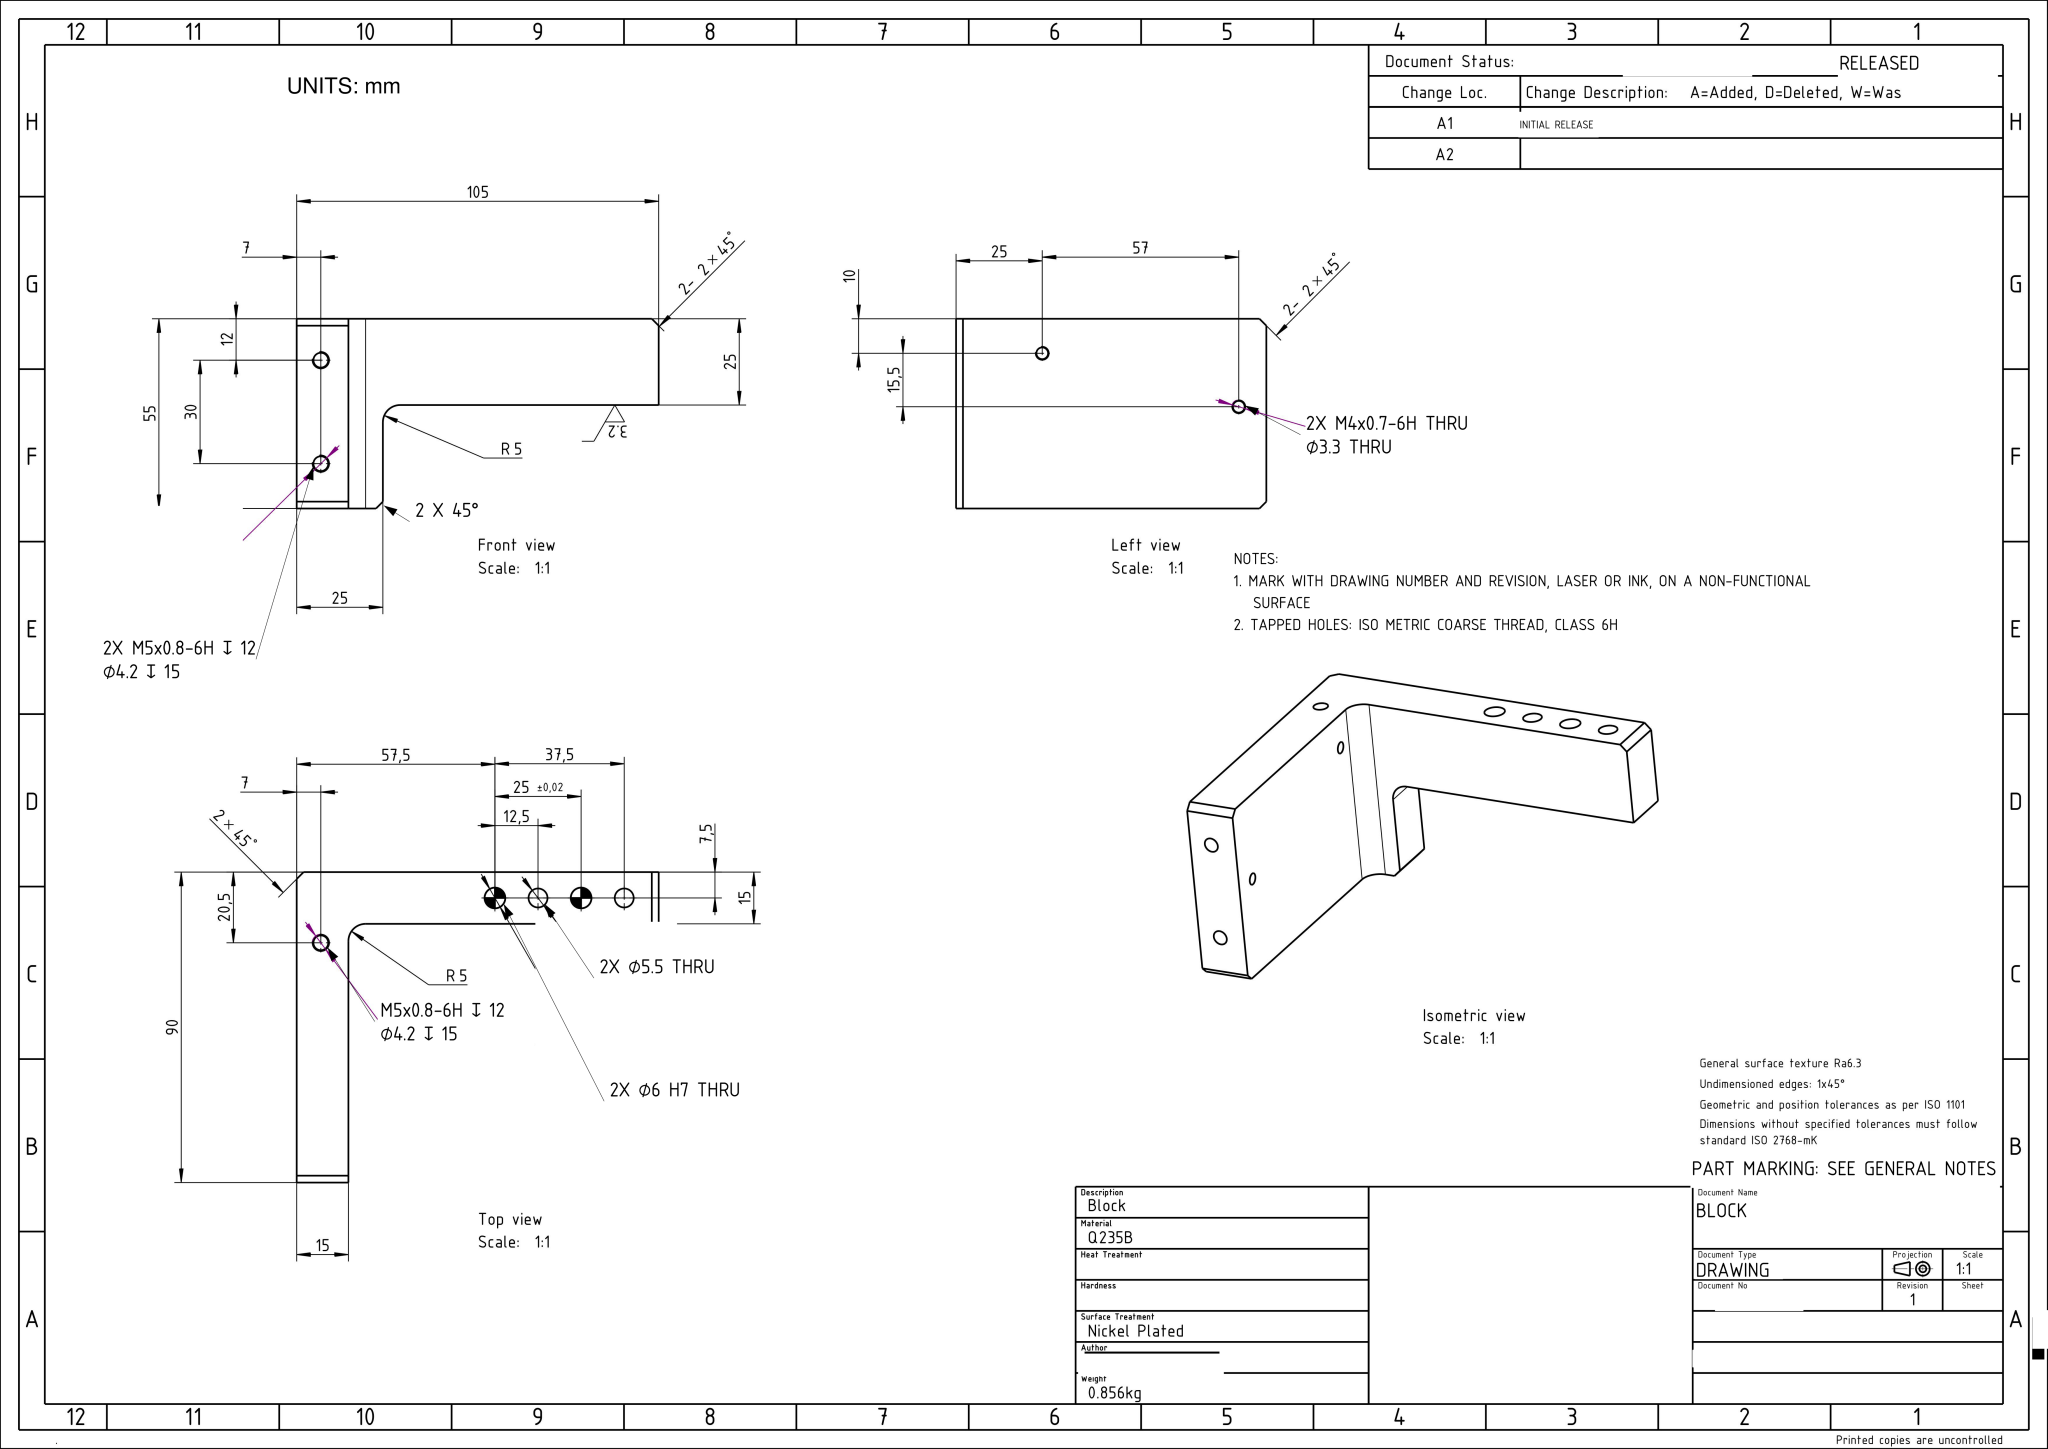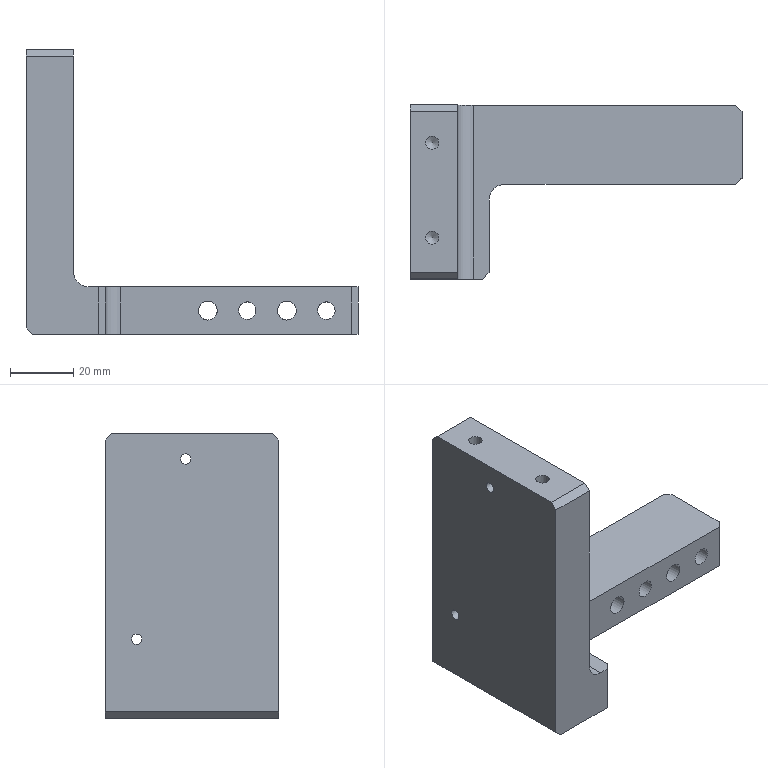Part | NX | mm | 1 solid | 30 faces | box 105 x 55 x 90 mm | volume 109116 mm3 | plane 16 | cylinder 11 | cone 3 | commonest cylinder face diameters 4.2 x3 6 x2 5.5 x2 10 x2 3.3 x2
STEP:
#1=CARTESIAN_POINT('',(0.,0.,0.));
#2=DIRECTION('',(0.,0.,1.));
#3=DIRECTION('',(1.,0.,0.));
#4=AXIS2_PLACEMENT_3D('',#1,#2,#3);
#5=(LENGTH_UNIT()NAMED_UNIT(*)SI_UNIT(.MILLI.,.METRE.));
#6=UNCERTAINTY_MEASURE_WITH_UNIT(LENGTH_MEASURE(0.00002),#5,'','');
#7=(NAMED_UNIT(*)PLANE_ANGLE_UNIT()SI_UNIT($,.RADIAN.));
#8=PLANE_ANGLE_MEASURE_WITH_UNIT(PLANE_ANGLE_MEASURE(0.01745),#7);
#9=DIMENSIONAL_EXPONENTS(0.,0.,0.,0.,0.,0.,0.);
#10=(CONVERSION_BASED_UNIT('',#8)NAMED_UNIT(#9)PLANE_ANGLE_UNIT());
#11=(NAMED_UNIT(*)SI_UNIT($,.STERADIAN.)SOLID_ANGLE_UNIT());
#12=(GEOMETRIC_REPRESENTATION_CONTEXT(3)GLOBAL_UNCERTAINTY_ASSIGNED_CONTEXT((#6))GLOBAL_UNIT_ASSIGNED_CONTEXT((#5,#10,#11))REPRESENTATION_CONTEXT('',''));
#13=SHAPE_REPRESENTATION('',(#4),#12);
#14=CARTESIAN_POINT('',(-32.5,-30.,15.));
#15=VERTEX_POINT('',#14);
#16=CARTESIAN_POINT('',(-29.5,-30.,15.));
#17=VERTEX_POINT('',#16);
#18=CARTESIAN_POINT('',(-52.5,-30.,15.));
#19=DIRECTION('',(1.,-0.,0.));
#20=VECTOR('',#19,1.);
#21=LINE('',#18,#20);
#22=EDGE_CURVE('',#15,#17,#21,.T.);
#23=ORIENTED_EDGE('',*,*,#22,.T.);
#24=CARTESIAN_POINT('',(-27.5,-28.,15.));
#25=VERTEX_POINT('',#24);
#26=CARTESIAN_POINT('',(0.25,-0.25,15.));
#27=DIRECTION('',(0.7071,0.7071,0.));
#28=VECTOR('',#27,1.);
#29=LINE('',#26,#28);
#30=EDGE_CURVE('',#17,#25,#29,.T.);
#31=ORIENTED_EDGE('',*,*,#30,.T.);
#32=CARTESIAN_POINT('',(-27.5,-5.,15.));
#33=VERTEX_POINT('',#32);
#34=CARTESIAN_POINT('',(-27.5,-30.,15.));
#35=DIRECTION('',(0.,1.,0.));
#36=VECTOR('',#35,1.);
#37=LINE('',#34,#36);
#38=EDGE_CURVE('',#25,#33,#37,.T.);
#39=ORIENTED_EDGE('',*,*,#38,.T.);
#40=CARTESIAN_POINT('',(-22.5,0.,15.));
#41=VERTEX_POINT('',#40);
#42=CARTESIAN_POINT('',(-22.5,-5.,15.));
#43=DIRECTION('',(0.,0.,-1.));
#44=DIRECTION('',(1.,0.,0.));
#45=AXIS2_PLACEMENT_3D('',#42,#43,#44);
#46=CIRCLE('',#45,5.);
#47=EDGE_CURVE('',#33,#41,#46,.T.);
#48=ORIENTED_EDGE('',*,*,#47,.T.);
#49=CARTESIAN_POINT('',(50.5,-0.,15.));
#50=VERTEX_POINT('',#49);
#51=CARTESIAN_POINT('',(-27.5,0.,15.));
#52=DIRECTION('',(1.,-0.,0.));
#53=VECTOR('',#52,1.);
#54=LINE('',#51,#53);
#55=EDGE_CURVE('',#41,#50,#54,.T.);
#56=ORIENTED_EDGE('',*,*,#55,.T.);
#57=CARTESIAN_POINT('',(52.5,2.,15.));
#58=VERTEX_POINT('',#57);
#59=CARTESIAN_POINT('',(25.25,-25.25,15.));
#60=DIRECTION('',(0.7071,0.7071,0.));
#61=VECTOR('',#60,1.);
#62=LINE('',#59,#61);
#63=EDGE_CURVE('',#50,#58,#62,.T.);
#64=ORIENTED_EDGE('',*,*,#63,.T.);
#65=CARTESIAN_POINT('',(52.5,23.,15.));
#66=VERTEX_POINT('',#65);
#67=CARTESIAN_POINT('',(52.5,-0.,15.));
#68=DIRECTION('',(0.,1.,0.));
#69=VECTOR('',#68,1.);
#70=LINE('',#67,#69);
#71=EDGE_CURVE('',#58,#66,#70,.T.);
#72=ORIENTED_EDGE('',*,*,#71,.T.);
#73=CARTESIAN_POINT('',(50.5,25.,15.));
#74=VERTEX_POINT('',#73);
#75=CARTESIAN_POINT('',(37.75,37.75,15.));
#76=DIRECTION('',(-0.7071,0.7071,0.));
#77=VECTOR('',#76,1.);
#78=LINE('',#75,#77);
#79=EDGE_CURVE('',#66,#74,#78,.T.);
#80=ORIENTED_EDGE('',*,*,#79,.T.);
#81=CARTESIAN_POINT('',(-32.5,25.,15.));
#82=VERTEX_POINT('',#81);
#83=CARTESIAN_POINT('',(52.5,25.,15.));
#84=DIRECTION('',(-1.,0.,0.));
#85=VECTOR('',#84,1.);
#86=LINE('',#83,#85);
#87=EDGE_CURVE('',#74,#82,#86,.T.);
#88=ORIENTED_EDGE('',*,*,#87,.T.);
#89=CARTESIAN_POINT('',(-32.5,0.,15.));
#90=DIRECTION('',(-0.,-1.,0.));
#91=VECTOR('',#90,1.);
#92=LINE('',#89,#91);
#93=EDGE_CURVE('',#82,#15,#92,.T.);
#94=ORIENTED_EDGE('',*,*,#93,.T.);
#95=EDGE_LOOP('',(#23,#31,#39,#48,#56,#64,#72,#80,#88,#94));
#96=FACE_OUTER_BOUND('',#95,.T.);
#97=CARTESIAN_POINT('',(0.,0.,15.));
#98=DIRECTION('',(0.,0.,1.));
#99=DIRECTION('',(1.,0.,0.));
#100=AXIS2_PLACEMENT_3D('',#97,#98,#99);
#101=PLANE('',#100);
#102=ADVANCED_FACE('',(#96),#101,.T.);
#103=CARTESIAN_POINT('',(-52.5,16.65,25.));
#104=VERTEX_POINT('',#103);
#105=CARTESIAN_POINT('',(-52.5,15.,25.));
#106=DIRECTION('',(1.,-0.,0.));
#107=DIRECTION('',(0.,1.,0.));
#108=AXIS2_PLACEMENT_3D('',#105,#106,#107);
#109=CIRCLE('',#108,1.65);
#110=EDGE_CURVE('',#104,#104,#109,.T.);
#111=ORIENTED_EDGE('',*,*,#110,.T.);
#112=EDGE_LOOP('',(#111));
#113=FACE_BOUND('',#112,.T.);
#114=CARTESIAN_POINT('',(-52.5,1.15,82.));
#115=VERTEX_POINT('',#114);
#116=CARTESIAN_POINT('',(-52.5,-0.5,82.));
#117=DIRECTION('',(1.,-0.,0.));
#118=DIRECTION('',(0.,1.,0.));
#119=AXIS2_PLACEMENT_3D('',#116,#117,#118);
#120=CIRCLE('',#119,1.65);
#121=EDGE_CURVE('',#115,#115,#120,.T.);
#122=ORIENTED_EDGE('',*,*,#121,.T.);
#123=EDGE_LOOP('',(#122));
#124=FACE_BOUND('',#123,.T.);
#125=CARTESIAN_POINT('',(-52.5,25.,88.));
#126=VERTEX_POINT('',#125);
#127=CARTESIAN_POINT('',(-52.5,25.,2.));
#128=VERTEX_POINT('',#127);
#129=CARTESIAN_POINT('',(-52.5,25.,15.));
#130=DIRECTION('',(0.,0.,-1.));
#131=VECTOR('',#130,1.);
#132=LINE('',#129,#131);
#133=EDGE_CURVE('',#126,#128,#132,.T.);
#134=ORIENTED_EDGE('',*,*,#133,.T.);
#135=CARTESIAN_POINT('',(-52.5,-30.,2.));
#136=VERTEX_POINT('',#135);
#137=CARTESIAN_POINT('',(-52.5,25.,2.));
#138=DIRECTION('',(-0.,-1.,0.));
#139=VECTOR('',#138,1.);
#140=LINE('',#137,#139);
#141=EDGE_CURVE('',#128,#136,#140,.T.);
#142=ORIENTED_EDGE('',*,*,#141,.T.);
#143=CARTESIAN_POINT('',(-52.5,-30.,88.));
#144=VERTEX_POINT('',#143);
#145=CARTESIAN_POINT('',(-52.5,-30.,15.));
#146=DIRECTION('',(0.,0.,-1.));
#147=VECTOR('',#146,1.);
#148=LINE('',#145,#147);
#149=EDGE_CURVE('',#144,#136,#148,.T.);
#150=ORIENTED_EDGE('',*,*,#149,.F.);
#151=CARTESIAN_POINT('',(-52.5,-28.,90.));
#152=VERTEX_POINT('',#151);
#153=CARTESIAN_POINT('',(-52.5,-28.,90.));
#154=DIRECTION('',(0.,0.7071,0.7071));
#155=VECTOR('',#154,1.);
#156=LINE('',#153,#155);
#157=EDGE_CURVE('',#144,#152,#156,.T.);
#158=ORIENTED_EDGE('',*,*,#157,.T.);
#159=CARTESIAN_POINT('',(-52.5,23.,90.));
#160=VERTEX_POINT('',#159);
#161=CARTESIAN_POINT('',(-52.5,25.,90.));
#162=DIRECTION('',(-0.,-1.,0.));
#163=VECTOR('',#162,1.);
#164=LINE('',#161,#163);
#165=EDGE_CURVE('',#160,#152,#164,.T.);
#166=ORIENTED_EDGE('',*,*,#165,.F.);
#167=CARTESIAN_POINT('',(-52.5,25.,88.));
#168=DIRECTION('',(0.,0.7071,-0.7071));
#169=VECTOR('',#168,1.);
#170=LINE('',#167,#169);
#171=EDGE_CURVE('',#160,#126,#170,.T.);
#172=ORIENTED_EDGE('',*,*,#171,.T.);
#173=EDGE_LOOP('',(#134,#142,#150,#158,#166,#172));
#174=FACE_BOUND('',#173,.T.);
#175=CARTESIAN_POINT('',(-52.5,25.,15.));
#176=DIRECTION('',(1.,-0.,0.));
#177=DIRECTION('',(0.,1.,0.));
#178=AXIS2_PLACEMENT_3D('',#175,#176,#177);
#179=PLANE('',#178);
#180=ADVANCED_FACE('',(#113,#124,#174),#179,.F.);
#181=CARTESIAN_POINT('',(-50.5,-30.,0.));
#182=VERTEX_POINT('',#181);
#183=CARTESIAN_POINT('',(-29.5,-30.,0.));
#184=VERTEX_POINT('',#183);
#185=CARTESIAN_POINT('',(-52.5,-30.,0.));
#186=DIRECTION('',(1.,-0.,0.));
#187=VECTOR('',#186,1.);
#188=LINE('',#185,#187);
#189=EDGE_CURVE('',#182,#184,#188,.T.);
#190=ORIENTED_EDGE('',*,*,#189,.T.);
#191=CARTESIAN_POINT('',(-29.5,-30.,15.));
#192=DIRECTION('',(0.,0.,1.));
#193=VECTOR('',#192,1.);
#194=LINE('',#191,#193);
#195=EDGE_CURVE('',#184,#17,#194,.T.);
#196=ORIENTED_EDGE('',*,*,#195,.T.);
#197=ORIENTED_EDGE('',*,*,#22,.F.);
#198=CARTESIAN_POINT('',(-37.5,-30.,20.));
#199=VERTEX_POINT('',#198);
#200=CARTESIAN_POINT('',(-32.5,-30.,20.));
#201=DIRECTION('',(0.,1.,0.));
#202=DIRECTION('',(-1.,0.,0.));
#203=AXIS2_PLACEMENT_3D('',#200,#201,#202);
#204=CIRCLE('',#203,5.);
#205=EDGE_CURVE('',#15,#199,#204,.T.);
#206=ORIENTED_EDGE('',*,*,#205,.T.);
#207=CARTESIAN_POINT('',(-37.5,-30.,88.));
#208=VERTEX_POINT('',#207);
#209=CARTESIAN_POINT('',(-37.5,-30.,15.));
#210=DIRECTION('',(0.,0.,1.));
#211=VECTOR('',#210,1.);
#212=LINE('',#209,#211);
#213=EDGE_CURVE('',#199,#208,#212,.T.);
#214=ORIENTED_EDGE('',*,*,#213,.T.);
#215=CARTESIAN_POINT('',(-52.5,-30.,88.));
#216=DIRECTION('',(-1.,0.,0.));
#217=VECTOR('',#216,1.);
#218=LINE('',#215,#217);
#219=EDGE_CURVE('',#208,#144,#218,.T.);
#220=ORIENTED_EDGE('',*,*,#219,.T.);
#221=ORIENTED_EDGE('',*,*,#149,.T.);
#222=CARTESIAN_POINT('',(-52.5,-30.,2.));
#223=DIRECTION('',(0.7071,-0.,-0.7071));
#224=VECTOR('',#223,1.);
#225=LINE('',#222,#224);
#226=EDGE_CURVE('',#136,#182,#225,.T.);
#227=ORIENTED_EDGE('',*,*,#226,.T.);
#228=EDGE_LOOP('',(#190,#196,#197,#206,#214,#220,#221,#227));
#229=FACE_OUTER_BOUND('',#228,.T.);
#230=CARTESIAN_POINT('',(-52.5,-30.,15.));
#231=DIRECTION('',(0.,1.,0.));
#232=DIRECTION('',(-1.,0.,0.));
#233=AXIS2_PLACEMENT_3D('',#230,#231,#232);
#234=PLANE('',#233);
#235=ADVANCED_FACE('',(#229),#234,.F.);
#236=ORIENTED_EDGE('',*,*,#38,.F.);
#237=CARTESIAN_POINT('',(-27.5,-28.,0.));
#238=VERTEX_POINT('',#237);
#239=CARTESIAN_POINT('',(-27.5,-28.,15.));
#240=DIRECTION('',(0.,0.,-1.));
#241=VECTOR('',#240,1.);
#242=LINE('',#239,#241);
#243=EDGE_CURVE('',#25,#238,#242,.T.);
#244=ORIENTED_EDGE('',*,*,#243,.T.);
#245=CARTESIAN_POINT('',(-27.5,-5.,0.));
#246=VERTEX_POINT('',#245);
#247=CARTESIAN_POINT('',(-27.5,-30.,0.));
#248=DIRECTION('',(0.,1.,0.));
#249=VECTOR('',#248,1.);
#250=LINE('',#247,#249);
#251=EDGE_CURVE('',#238,#246,#250,.T.);
#252=ORIENTED_EDGE('',*,*,#251,.T.);
#253=CARTESIAN_POINT('',(-27.5,-5.,15.));
#254=DIRECTION('',(0.,0.,1.));
#255=VECTOR('',#254,1.);
#256=LINE('',#253,#255);
#257=EDGE_CURVE('',#246,#33,#256,.T.);
#258=ORIENTED_EDGE('',*,*,#257,.T.);
#259=EDGE_LOOP('',(#236,#244,#252,#258));
#260=FACE_OUTER_BOUND('',#259,.T.);
#261=CARTESIAN_POINT('',(-27.5,-30.,15.));
#262=DIRECTION('',(-1.,0.,0.));
#263=DIRECTION('',(0.,0.,1.));
#264=AXIS2_PLACEMENT_3D('',#261,#262,#263);
#265=PLANE('',#264);
#266=ADVANCED_FACE('',(#260),#265,.F.);
#267=CARTESIAN_POINT('',(39.75,-0.,7.5));
#268=VERTEX_POINT('',#267);
#269=CARTESIAN_POINT('',(42.5,-0.,7.5));
#270=DIRECTION('',(0.,1.,0.));
#271=DIRECTION('',(-1.,0.,0.));
#272=AXIS2_PLACEMENT_3D('',#269,#270,#271);
#273=CIRCLE('',#272,2.75);
#274=EDGE_CURVE('',#268,#268,#273,.T.);
#275=ORIENTED_EDGE('',*,*,#274,.T.);
#276=EDGE_LOOP('',(#275));
#277=FACE_BOUND('',#276,.T.);
#278=CARTESIAN_POINT('',(14.75,-0.,7.5));
#279=VERTEX_POINT('',#278);
#280=CARTESIAN_POINT('',(17.5,-0.,7.5));
#281=DIRECTION('',(0.,1.,0.));
#282=DIRECTION('',(-1.,0.,0.));
#283=AXIS2_PLACEMENT_3D('',#280,#281,#282);
#284=CIRCLE('',#283,2.75);
#285=EDGE_CURVE('',#279,#279,#284,.T.);
#286=ORIENTED_EDGE('',*,*,#285,.T.);
#287=EDGE_LOOP('',(#286));
#288=FACE_BOUND('',#287,.T.);
#289=CARTESIAN_POINT('',(27.,-0.,7.5));
#290=VERTEX_POINT('',#289);
#291=CARTESIAN_POINT('',(30.,-0.,7.5));
#292=DIRECTION('',(0.,1.,0.));
#293=DIRECTION('',(-1.,0.,0.));
#294=AXIS2_PLACEMENT_3D('',#291,#292,#293);
#295=CIRCLE('',#294,3.);
#296=EDGE_CURVE('',#290,#290,#295,.T.);
#297=ORIENTED_EDGE('',*,*,#296,.T.);
#298=EDGE_LOOP('',(#297));
#299=FACE_BOUND('',#298,.T.);
#300=CARTESIAN_POINT('',(2.,-0.,7.5));
#301=VERTEX_POINT('',#300);
#302=CARTESIAN_POINT('',(5.,-0.,7.5));
#303=DIRECTION('',(0.,1.,0.));
#304=DIRECTION('',(-1.,0.,0.));
#305=AXIS2_PLACEMENT_3D('',#302,#303,#304);
#306=CIRCLE('',#305,3.);
#307=EDGE_CURVE('',#301,#301,#306,.T.);
#308=ORIENTED_EDGE('',*,*,#307,.T.);
#309=EDGE_LOOP('',(#308));
#310=FACE_BOUND('',#309,.T.);
#311=CARTESIAN_POINT('',(-22.5,0.,0.));
#312=VERTEX_POINT('',#311);
#313=CARTESIAN_POINT('',(50.5,-0.,0.));
#314=VERTEX_POINT('',#313);
#315=CARTESIAN_POINT('',(-27.5,0.,0.));
#316=DIRECTION('',(1.,-0.,0.));
#317=VECTOR('',#316,1.);
#318=LINE('',#315,#317);
#319=EDGE_CURVE('',#312,#314,#318,.T.);
#320=ORIENTED_EDGE('',*,*,#319,.T.);
#321=CARTESIAN_POINT('',(50.5,-0.,15.));
#322=DIRECTION('',(0.,0.,1.));
#323=VECTOR('',#322,1.);
#324=LINE('',#321,#323);
#325=EDGE_CURVE('',#314,#50,#324,.T.);
#326=ORIENTED_EDGE('',*,*,#325,.T.);
#327=ORIENTED_EDGE('',*,*,#55,.F.);
#328=CARTESIAN_POINT('',(-22.5,0.,0.));
#329=DIRECTION('',(0.,0.,-1.));
#330=VECTOR('',#329,1.);
#331=LINE('',#328,#330);
#332=EDGE_CURVE('',#41,#312,#331,.T.);
#333=ORIENTED_EDGE('',*,*,#332,.T.);
#334=EDGE_LOOP('',(#320,#326,#327,#333));
#335=FACE_BOUND('',#334,.T.);
#336=CARTESIAN_POINT('',(-27.5,0.,15.));
#337=DIRECTION('',(0.,1.,0.));
#338=DIRECTION('',(-1.,0.,0.));
#339=AXIS2_PLACEMENT_3D('',#336,#337,#338);
#340=PLANE('',#339);
#341=ADVANCED_FACE('',(#277,#288,#299,#310,#335),#340,.F.);
#342=CARTESIAN_POINT('',(52.5,2.,0.));
#343=VERTEX_POINT('',#342);
#344=CARTESIAN_POINT('',(52.5,23.,0.));
#345=VERTEX_POINT('',#344);
#346=CARTESIAN_POINT('',(52.5,-0.,0.));
#347=DIRECTION('',(0.,1.,0.));
#348=VECTOR('',#347,1.);
#349=LINE('',#346,#348);
#350=EDGE_CURVE('',#343,#345,#349,.T.);
#351=ORIENTED_EDGE('',*,*,#350,.T.);
#352=CARTESIAN_POINT('',(52.5,23.,15.));
#353=DIRECTION('',(0.,0.,1.));
#354=VECTOR('',#353,1.);
#355=LINE('',#352,#354);
#356=EDGE_CURVE('',#345,#66,#355,.T.);
#357=ORIENTED_EDGE('',*,*,#356,.T.);
#358=ORIENTED_EDGE('',*,*,#71,.F.);
#359=CARTESIAN_POINT('',(52.5,2.,15.));
#360=DIRECTION('',(0.,0.,-1.));
#361=VECTOR('',#360,1.);
#362=LINE('',#359,#361);
#363=EDGE_CURVE('',#58,#343,#362,.T.);
#364=ORIENTED_EDGE('',*,*,#363,.T.);
#365=EDGE_LOOP('',(#351,#357,#358,#364));
#366=FACE_OUTER_BOUND('',#365,.T.);
#367=CARTESIAN_POINT('',(52.5,-0.,15.));
#368=DIRECTION('',(-1.,0.,0.));
#369=DIRECTION('',(0.,0.,1.));
#370=AXIS2_PLACEMENT_3D('',#367,#368,#369);
#371=PLANE('',#370);
#372=ADVANCED_FACE('',(#366),#371,.F.);
#373=CARTESIAN_POINT('',(42.5,25.,4.75));
#374=VERTEX_POINT('',#373);
#375=CARTESIAN_POINT('',(42.5,25.,7.5));
#376=DIRECTION('',(0.,-1.,0.));
#377=DIRECTION('',(0.,0.,-1.));
#378=AXIS2_PLACEMENT_3D('',#375,#376,#377);
#379=CIRCLE('',#378,2.75);
#380=EDGE_CURVE('',#374,#374,#379,.T.);
#381=ORIENTED_EDGE('',*,*,#380,.T.);
#382=EDGE_LOOP('',(#381));
#383=FACE_BOUND('',#382,.T.);
#384=CARTESIAN_POINT('',(17.5,25.,4.75));
#385=VERTEX_POINT('',#384);
#386=CARTESIAN_POINT('',(17.5,25.,7.5));
#387=DIRECTION('',(0.,-1.,0.));
#388=DIRECTION('',(0.,0.,-1.));
#389=AXIS2_PLACEMENT_3D('',#386,#387,#388);
#390=CIRCLE('',#389,2.75);
#391=EDGE_CURVE('',#385,#385,#390,.T.);
#392=ORIENTED_EDGE('',*,*,#391,.T.);
#393=EDGE_LOOP('',(#392));
#394=FACE_BOUND('',#393,.T.);
#395=CARTESIAN_POINT('',(30.,25.,4.5));
#396=VERTEX_POINT('',#395);
#397=CARTESIAN_POINT('',(30.,25.,7.5));
#398=DIRECTION('',(0.,-1.,0.));
#399=DIRECTION('',(0.,0.,-1.));
#400=AXIS2_PLACEMENT_3D('',#397,#398,#399);
#401=CIRCLE('',#400,3.);
#402=EDGE_CURVE('',#396,#396,#401,.T.);
#403=ORIENTED_EDGE('',*,*,#402,.T.);
#404=EDGE_LOOP('',(#403));
#405=FACE_BOUND('',#404,.T.);
#406=CARTESIAN_POINT('',(5.,25.,4.5));
#407=VERTEX_POINT('',#406);
#408=CARTESIAN_POINT('',(5.,25.,7.5));
#409=DIRECTION('',(0.,-1.,0.));
#410=DIRECTION('',(0.,0.,-1.));
#411=AXIS2_PLACEMENT_3D('',#408,#409,#410);
#412=CIRCLE('',#411,3.);
#413=EDGE_CURVE('',#407,#407,#412,.T.);
#414=ORIENTED_EDGE('',*,*,#413,.T.);
#415=EDGE_LOOP('',(#414));
#416=FACE_BOUND('',#415,.T.);
#417=CARTESIAN_POINT('',(-45.5,25.,18.4));
#418=VERTEX_POINT('',#417);
#419=CARTESIAN_POINT('',(-45.5,25.,20.5));
#420=DIRECTION('',(0.,-1.,0.));
#421=DIRECTION('',(0.,0.,-1.));
#422=AXIS2_PLACEMENT_3D('',#419,#420,#421);
#423=CIRCLE('',#422,2.1);
#424=EDGE_CURVE('',#418,#418,#423,.T.);
#425=ORIENTED_EDGE('',*,*,#424,.T.);
#426=EDGE_LOOP('',(#425));
#427=FACE_BOUND('',#426,.T.);
#428=CARTESIAN_POINT('',(50.5,25.,0.));
#429=VERTEX_POINT('',#428);
#430=CARTESIAN_POINT('',(-50.5,25.,0.));
#431=VERTEX_POINT('',#430);
#432=CARTESIAN_POINT('',(52.5,25.,0.));
#433=DIRECTION('',(-1.,0.,0.));
#434=VECTOR('',#433,1.);
#435=LINE('',#432,#434);
#436=EDGE_CURVE('',#429,#431,#435,.T.);
#437=ORIENTED_EDGE('',*,*,#436,.T.);
#438=CARTESIAN_POINT('',(-52.5,25.,2.));
#439=DIRECTION('',(-0.7071,0.,0.7071));
#440=VECTOR('',#439,1.);
#441=LINE('',#438,#440);
#442=EDGE_CURVE('',#431,#128,#441,.T.);
#443=ORIENTED_EDGE('',*,*,#442,.T.);
#444=ORIENTED_EDGE('',*,*,#133,.F.);
#445=CARTESIAN_POINT('',(-37.5,25.,88.));
#446=VERTEX_POINT('',#445);
#447=CARTESIAN_POINT('',(52.5,25.,88.));
#448=DIRECTION('',(1.,0.,0.));
#449=VECTOR('',#448,1.);
#450=LINE('',#447,#449);
#451=EDGE_CURVE('',#126,#446,#450,.T.);
#452=ORIENTED_EDGE('',*,*,#451,.T.);
#453=CARTESIAN_POINT('',(-37.5,25.,20.));
#454=VERTEX_POINT('',#453);
#455=CARTESIAN_POINT('',(-37.5,25.,15.));
#456=DIRECTION('',(0.,0.,1.));
#457=VECTOR('',#456,1.);
#458=LINE('',#455,#457);
#459=EDGE_CURVE('',#454,#446,#458,.T.);
#460=ORIENTED_EDGE('',*,*,#459,.F.);
#461=CARTESIAN_POINT('',(-32.5,25.,20.));
#462=DIRECTION('',(0.,-1.,0.));
#463=DIRECTION('',(0.,0.,-1.));
#464=AXIS2_PLACEMENT_3D('',#461,#462,#463);
#465=CIRCLE('',#464,5.);
#466=EDGE_CURVE('',#454,#82,#465,.T.);
#467=ORIENTED_EDGE('',*,*,#466,.T.);
#468=ORIENTED_EDGE('',*,*,#87,.F.);
#469=CARTESIAN_POINT('',(50.5,25.,15.));
#470=DIRECTION('',(0.,0.,-1.));
#471=VECTOR('',#470,1.);
#472=LINE('',#469,#471);
#473=EDGE_CURVE('',#74,#429,#472,.T.);
#474=ORIENTED_EDGE('',*,*,#473,.T.);
#475=EDGE_LOOP('',(#437,#443,#444,#452,#460,#467,#468,#474));
#476=FACE_BOUND('',#475,.T.);
#477=CARTESIAN_POINT('',(52.5,25.,15.));
#478=DIRECTION('',(0.,-1.,0.));
#479=DIRECTION('',(0.,0.,-1.));
#480=AXIS2_PLACEMENT_3D('',#477,#478,#479);
#481=PLANE('',#480);
#482=ADVANCED_FACE('',(#383,#394,#405,#416,#427,#476),#481,.F.);
#483=ORIENTED_EDGE('',*,*,#251,.F.);
#484=CARTESIAN_POINT('',(-27.5,-28.,0.));
#485=DIRECTION('',(-0.7071,-0.7071,0.));
#486=VECTOR('',#485,1.);
#487=LINE('',#484,#486);
#488=EDGE_CURVE('',#238,#184,#487,.T.);
#489=ORIENTED_EDGE('',*,*,#488,.T.);
#490=ORIENTED_EDGE('',*,*,#189,.F.);
#491=CARTESIAN_POINT('',(-50.5,0.,0.));
#492=DIRECTION('',(0.,1.,0.));
#493=VECTOR('',#492,1.);
#494=LINE('',#491,#493);
#495=EDGE_CURVE('',#182,#431,#494,.T.);
#496=ORIENTED_EDGE('',*,*,#495,.T.);
#497=ORIENTED_EDGE('',*,*,#436,.F.);
#498=CARTESIAN_POINT('',(50.5,25.,0.));
#499=DIRECTION('',(0.7071,-0.7071,0.));
#500=VECTOR('',#499,1.);
#501=LINE('',#498,#500);
#502=EDGE_CURVE('',#429,#345,#501,.T.);
#503=ORIENTED_EDGE('',*,*,#502,.T.);
#504=ORIENTED_EDGE('',*,*,#350,.F.);
#505=CARTESIAN_POINT('',(52.5,2.,0.));
#506=DIRECTION('',(-0.7071,-0.7071,0.));
#507=VECTOR('',#506,1.);
#508=LINE('',#505,#507);
#509=EDGE_CURVE('',#343,#314,#508,.T.);
#510=ORIENTED_EDGE('',*,*,#509,.T.);
#511=ORIENTED_EDGE('',*,*,#319,.F.);
#512=CARTESIAN_POINT('',(-22.5,-5.,0.));
#513=DIRECTION('',(0.,0.,1.));
#514=DIRECTION('',(1.,0.,0.));
#515=AXIS2_PLACEMENT_3D('',#512,#513,#514);
#516=CIRCLE('',#515,5.);
#517=EDGE_CURVE('',#312,#246,#516,.T.);
#518=ORIENTED_EDGE('',*,*,#517,.T.);
#519=EDGE_LOOP('',(#483,#489,#490,#496,#497,#503,#504,#510,#511,#518));
#520=FACE_OUTER_BOUND('',#519,.T.);
#521=CARTESIAN_POINT('',(0.,0.,0.));
#522=DIRECTION('',(0.,0.,1.));
#523=DIRECTION('',(1.,0.,0.));
#524=AXIS2_PLACEMENT_3D('',#521,#522,#523);
#525=PLANE('',#524);
#526=ADVANCED_FACE('',(#520),#525,.F.);
#527=CARTESIAN_POINT('',(-47.6,13.,90.));
#528=VERTEX_POINT('',#527);
#529=CARTESIAN_POINT('',(-45.5,13.,90.));
#530=DIRECTION('',(0.,0.,-1.));
#531=DIRECTION('',(-1.,0.,0.));
#532=AXIS2_PLACEMENT_3D('',#529,#530,#531);
#533=CIRCLE('',#532,2.1);
#534=EDGE_CURVE('',#528,#528,#533,.T.);
#535=ORIENTED_EDGE('',*,*,#534,.T.);
#536=EDGE_LOOP('',(#535));
#537=FACE_BOUND('',#536,.T.);
#538=CARTESIAN_POINT('',(-47.6,-17.,90.));
#539=VERTEX_POINT('',#538);
#540=CARTESIAN_POINT('',(-45.5,-17.,90.));
#541=DIRECTION('',(0.,0.,-1.));
#542=DIRECTION('',(-1.,0.,0.));
#543=AXIS2_PLACEMENT_3D('',#540,#541,#542);
#544=CIRCLE('',#543,2.1);
#545=EDGE_CURVE('',#539,#539,#544,.T.);
#546=ORIENTED_EDGE('',*,*,#545,.T.);
#547=EDGE_LOOP('',(#546));
#548=FACE_BOUND('',#547,.T.);
#549=CARTESIAN_POINT('',(-37.5,23.,90.));
#550=VERTEX_POINT('',#549);
#551=CARTESIAN_POINT('',(-37.5,-28.,90.));
#552=VERTEX_POINT('',#551);
#553=CARTESIAN_POINT('',(-37.5,25.,90.));
#554=DIRECTION('',(-0.,-1.,0.));
#555=VECTOR('',#554,1.);
#556=LINE('',#553,#555);
#557=EDGE_CURVE('',#550,#552,#556,.T.);
#558=ORIENTED_EDGE('',*,*,#557,.F.);
#559=CARTESIAN_POINT('',(-52.5,23.,90.));
#560=DIRECTION('',(-1.,0.,0.));
#561=VECTOR('',#560,1.);
#562=LINE('',#559,#561);
#563=EDGE_CURVE('',#550,#160,#562,.T.);
#564=ORIENTED_EDGE('',*,*,#563,.T.);
#565=ORIENTED_EDGE('',*,*,#165,.T.);
#566=CARTESIAN_POINT('',(-52.5,-28.,90.));
#567=DIRECTION('',(1.,-0.,0.));
#568=VECTOR('',#567,1.);
#569=LINE('',#566,#568);
#570=EDGE_CURVE('',#152,#552,#569,.T.);
#571=ORIENTED_EDGE('',*,*,#570,.T.);
#572=EDGE_LOOP('',(#558,#564,#565,#571));
#573=FACE_BOUND('',#572,.T.);
#574=CARTESIAN_POINT('',(-52.5,25.,90.));
#575=DIRECTION('',(0.,0.,-1.));
#576=DIRECTION('',(-0.,-1.,0.));
#577=AXIS2_PLACEMENT_3D('',#574,#575,#576);
#578=PLANE('',#577);
#579=ADVANCED_FACE('',(#537,#548,#573),#578,.F.);
#580=CARTESIAN_POINT('',(-37.5,13.35,25.));
#581=VERTEX_POINT('',#580);
#582=CARTESIAN_POINT('',(-37.5,15.,25.));
#583=DIRECTION('',(-1.,0.,0.));
#584=DIRECTION('',(0.,-1.,0.));
#585=AXIS2_PLACEMENT_3D('',#582,#583,#584);
#586=CIRCLE('',#585,1.65);
#587=EDGE_CURVE('',#581,#581,#586,.T.);
#588=ORIENTED_EDGE('',*,*,#587,.T.);
#589=EDGE_LOOP('',(#588));
#590=FACE_BOUND('',#589,.T.);
#591=CARTESIAN_POINT('',(-37.5,-2.15,82.));
#592=VERTEX_POINT('',#591);
#593=CARTESIAN_POINT('',(-37.5,-0.5,82.));
#594=DIRECTION('',(-1.,0.,0.));
#595=DIRECTION('',(0.,-1.,0.));
#596=AXIS2_PLACEMENT_3D('',#593,#594,#595);
#597=CIRCLE('',#596,1.65);
#598=EDGE_CURVE('',#592,#592,#597,.T.);
#599=ORIENTED_EDGE('',*,*,#598,.T.);
#600=EDGE_LOOP('',(#599));
#601=FACE_BOUND('',#600,.T.);
#602=ORIENTED_EDGE('',*,*,#459,.T.);
#603=CARTESIAN_POINT('',(-37.5,25.,88.));
#604=DIRECTION('',(-0.,-0.7071,0.7071));
#605=VECTOR('',#604,1.);
#606=LINE('',#603,#605);
#607=EDGE_CURVE('',#446,#550,#606,.T.);
#608=ORIENTED_EDGE('',*,*,#607,.T.);
#609=ORIENTED_EDGE('',*,*,#557,.T.);
#610=CARTESIAN_POINT('',(-37.5,-28.,90.));
#611=DIRECTION('',(-0.,-0.7071,-0.7071));
#612=VECTOR('',#611,1.);
#613=LINE('',#610,#612);
#614=EDGE_CURVE('',#552,#208,#613,.T.);
#615=ORIENTED_EDGE('',*,*,#614,.T.);
#616=ORIENTED_EDGE('',*,*,#213,.F.);
#617=CARTESIAN_POINT('',(-37.5,25.,20.));
#618=DIRECTION('',(0.,1.,0.));
#619=VECTOR('',#618,1.);
#620=LINE('',#617,#619);
#621=EDGE_CURVE('',#199,#454,#620,.T.);
#622=ORIENTED_EDGE('',*,*,#621,.T.);
#623=EDGE_LOOP('',(#602,#608,#609,#615,#616,#622));
#624=FACE_BOUND('',#623,.T.);
#625=CARTESIAN_POINT('',(-37.5,25.,15.));
#626=DIRECTION('',(-1.,0.,0.));
#627=DIRECTION('',(-0.,-1.,0.));
#628=AXIS2_PLACEMENT_3D('',#625,#626,#627);
#629=PLANE('',#628);
#630=ADVANCED_FACE('',(#590,#601,#624),#629,.F.);
#631=CARTESIAN_POINT('',(-47.6,-17.,75.));
#632=VERTEX_POINT('',#631);
#633=CARTESIAN_POINT('',(-45.5,-17.,75.));
#634=DIRECTION('',(0.,0.,1.));
#635=DIRECTION('',(-1.,0.,0.));
#636=AXIS2_PLACEMENT_3D('',#633,#634,#635);
#637=CIRCLE('',#636,2.1);
#638=EDGE_CURVE('',#632,#632,#637,.T.);
#639=ORIENTED_EDGE('',*,*,#638,.T.);
#640=EDGE_LOOP('',(#639));
#641=FACE_BOUND('',#640,.T.);
#642=CARTESIAN_POINT('',(-45.5,-17.,73.738));
#643=VERTEX_POINT('',#642);
#644=VERTEX_LOOP('',#643);
#645=FACE_BOUND('',#644,.T.);
#646=CARTESIAN_POINT('',(-45.5,-17.,75.));
#647=DIRECTION('',(0.,0.,1.));
#648=DIRECTION('',(1.,0.,-0.));
#649=AXIS2_PLACEMENT_3D('',#646,#647,#648);
#650=CONICAL_SURFACE('',#649,2.1,59.);
#651=ADVANCED_FACE('',(#641,#645),#650,.F.);
#652=ORIENTED_EDGE('',*,*,#638,.F.);
#653=EDGE_LOOP('',(#652));
#654=FACE_BOUND('',#653,.T.);
#655=ORIENTED_EDGE('',*,*,#545,.F.);
#656=EDGE_LOOP('',(#655));
#657=FACE_BOUND('',#656,.T.);
#658=CARTESIAN_POINT('',(-45.5,-17.,90.));
#659=DIRECTION('',(0.,0.,-1.));
#660=DIRECTION('',(-1.,0.,0.));
#661=AXIS2_PLACEMENT_3D('',#658,#659,#660);
#662=CYLINDRICAL_SURFACE('',#661,2.1);
#663=ADVANCED_FACE('',(#654,#657),#662,.F.);
#664=CARTESIAN_POINT('',(-47.6,13.,75.));
#665=VERTEX_POINT('',#664);
#666=CARTESIAN_POINT('',(-45.5,13.,75.));
#667=DIRECTION('',(0.,0.,1.));
#668=DIRECTION('',(-1.,0.,0.));
#669=AXIS2_PLACEMENT_3D('',#666,#667,#668);
#670=CIRCLE('',#669,2.1);
#671=EDGE_CURVE('',#665,#665,#670,.T.);
#672=ORIENTED_EDGE('',*,*,#671,.T.);
#673=EDGE_LOOP('',(#672));
#674=FACE_BOUND('',#673,.T.);
#675=CARTESIAN_POINT('',(-45.5,13.,73.738));
#676=VERTEX_POINT('',#675);
#677=VERTEX_LOOP('',#676);
#678=FACE_BOUND('',#677,.T.);
#679=CARTESIAN_POINT('',(-45.5,13.,75.));
#680=DIRECTION('',(0.,0.,1.));
#681=DIRECTION('',(1.,0.,-0.));
#682=AXIS2_PLACEMENT_3D('',#679,#680,#681);
#683=CONICAL_SURFACE('',#682,2.1,59.);
#684=ADVANCED_FACE('',(#674,#678),#683,.F.);
#685=ORIENTED_EDGE('',*,*,#671,.F.);
#686=EDGE_LOOP('',(#685));
#687=FACE_BOUND('',#686,.T.);
#688=ORIENTED_EDGE('',*,*,#534,.F.);
#689=EDGE_LOOP('',(#688));
#690=FACE_BOUND('',#689,.T.);
#691=CARTESIAN_POINT('',(-45.5,13.,90.));
#692=DIRECTION('',(0.,0.,-1.));
#693=DIRECTION('',(-1.,0.,0.));
#694=AXIS2_PLACEMENT_3D('',#691,#692,#693);
#695=CYLINDRICAL_SURFACE('',#694,2.1);
#696=ADVANCED_FACE('',(#687,#690),#695,.F.);
#697=CARTESIAN_POINT('',(-45.5,10.,18.4));
#698=VERTEX_POINT('',#697);
#699=CARTESIAN_POINT('',(-45.5,10.,20.5));
#700=DIRECTION('',(0.,1.,0.));
#701=DIRECTION('',(0.,0.,-1.));
#702=AXIS2_PLACEMENT_3D('',#699,#700,#701);
#703=CIRCLE('',#702,2.1);
#704=EDGE_CURVE('',#698,#698,#703,.T.);
#705=ORIENTED_EDGE('',*,*,#704,.T.);
#706=EDGE_LOOP('',(#705));
#707=FACE_BOUND('',#706,.T.);
#708=CARTESIAN_POINT('',(-45.5,8.738,20.5));
#709=VERTEX_POINT('',#708);
#710=VERTEX_LOOP('',#709);
#711=FACE_BOUND('',#710,.T.);
#712=CARTESIAN_POINT('',(-45.5,10.,20.5));
#713=DIRECTION('',(0.,1.,0.));
#714=DIRECTION('',(0.,-0.,1.));
#715=AXIS2_PLACEMENT_3D('',#712,#713,#714);
#716=CONICAL_SURFACE('',#715,2.1,59.);
#717=ADVANCED_FACE('',(#707,#711),#716,.F.);
#718=ORIENTED_EDGE('',*,*,#704,.F.);
#719=EDGE_LOOP('',(#718));
#720=FACE_BOUND('',#719,.T.);
#721=ORIENTED_EDGE('',*,*,#424,.F.);
#722=EDGE_LOOP('',(#721));
#723=FACE_BOUND('',#722,.T.);
#724=CARTESIAN_POINT('',(-45.5,25.,20.5));
#725=DIRECTION('',(0.,-1.,0.));
#726=DIRECTION('',(0.,0.,-1.));
#727=AXIS2_PLACEMENT_3D('',#724,#725,#726);
#728=CYLINDRICAL_SURFACE('',#727,2.1);
#729=ADVANCED_FACE('',(#720,#723),#728,.F.);
#730=ORIENTED_EDGE('',*,*,#413,.F.);
#731=EDGE_LOOP('',(#730));
#732=FACE_BOUND('',#731,.T.);
#733=ORIENTED_EDGE('',*,*,#307,.F.);
#734=EDGE_LOOP('',(#733));
#735=FACE_BOUND('',#734,.T.);
#736=CARTESIAN_POINT('',(5.,25.,7.5));
#737=DIRECTION('',(0.,-1.,0.));
#738=DIRECTION('',(0.,0.,-1.));
#739=AXIS2_PLACEMENT_3D('',#736,#737,#738);
#740=CYLINDRICAL_SURFACE('',#739,3.);
#741=ADVANCED_FACE('',(#732,#735),#740,.F.);
#742=ORIENTED_EDGE('',*,*,#402,.F.);
#743=EDGE_LOOP('',(#742));
#744=FACE_BOUND('',#743,.T.);
#745=ORIENTED_EDGE('',*,*,#296,.F.);
#746=EDGE_LOOP('',(#745));
#747=FACE_BOUND('',#746,.T.);
#748=CARTESIAN_POINT('',(30.,25.,7.5));
#749=DIRECTION('',(0.,-1.,0.));
#750=DIRECTION('',(0.,0.,-1.));
#751=AXIS2_PLACEMENT_3D('',#748,#749,#750);
#752=CYLINDRICAL_SURFACE('',#751,3.);
#753=ADVANCED_FACE('',(#744,#747),#752,.F.);
#754=ORIENTED_EDGE('',*,*,#391,.F.);
#755=EDGE_LOOP('',(#754));
#756=FACE_BOUND('',#755,.T.);
#757=ORIENTED_EDGE('',*,*,#285,.F.);
#758=EDGE_LOOP('',(#757));
#759=FACE_BOUND('',#758,.T.);
#760=CARTESIAN_POINT('',(17.5,25.,7.5));
#761=DIRECTION('',(0.,-1.,0.));
#762=DIRECTION('',(0.,0.,-1.));
#763=AXIS2_PLACEMENT_3D('',#760,#761,#762);
#764=CYLINDRICAL_SURFACE('',#763,2.75);
#765=ADVANCED_FACE('',(#756,#759),#764,.F.);
#766=ORIENTED_EDGE('',*,*,#380,.F.);
#767=EDGE_LOOP('',(#766));
#768=FACE_BOUND('',#767,.T.);
#769=ORIENTED_EDGE('',*,*,#274,.F.);
#770=EDGE_LOOP('',(#769));
#771=FACE_BOUND('',#770,.T.);
#772=CARTESIAN_POINT('',(42.5,25.,7.5));
#773=DIRECTION('',(0.,-1.,0.));
#774=DIRECTION('',(0.,0.,-1.));
#775=AXIS2_PLACEMENT_3D('',#772,#773,#774);
#776=CYLINDRICAL_SURFACE('',#775,2.75);
#777=ADVANCED_FACE('',(#768,#771),#776,.F.);
#778=ORIENTED_EDGE('',*,*,#47,.F.);
#779=ORIENTED_EDGE('',*,*,#257,.F.);
#780=ORIENTED_EDGE('',*,*,#517,.F.);
#781=ORIENTED_EDGE('',*,*,#332,.F.);
#782=EDGE_LOOP('',(#778,#779,#780,#781));
#783=FACE_OUTER_BOUND('',#782,.T.);
#784=CARTESIAN_POINT('',(-22.5,-5.,15.));
#785=DIRECTION('',(0.,0.,1.));
#786=DIRECTION('',(1.,0.,0.));
#787=AXIS2_PLACEMENT_3D('',#784,#785,#786);
#788=CYLINDRICAL_SURFACE('',#787,5.);
#789=ADVANCED_FACE('',(#783),#788,.F.);
#790=ORIENTED_EDGE('',*,*,#466,.F.);
#791=ORIENTED_EDGE('',*,*,#621,.F.);
#792=ORIENTED_EDGE('',*,*,#205,.F.);
#793=ORIENTED_EDGE('',*,*,#93,.F.);
#794=EDGE_LOOP('',(#790,#791,#792,#793));
#795=FACE_OUTER_BOUND('',#794,.T.);
#796=CARTESIAN_POINT('',(-32.5,0.,20.));
#797=DIRECTION('',(-0.,-1.,0.));
#798=DIRECTION('',(1.,-0.,0.));
#799=AXIS2_PLACEMENT_3D('',#796,#797,#798);
#800=CYLINDRICAL_SURFACE('',#799,5.);
#801=ADVANCED_FACE('',(#795),#800,.F.);
#802=ORIENTED_EDGE('',*,*,#121,.F.);
#803=EDGE_LOOP('',(#802));
#804=FACE_BOUND('',#803,.T.);
#805=ORIENTED_EDGE('',*,*,#598,.F.);
#806=EDGE_LOOP('',(#805));
#807=FACE_BOUND('',#806,.T.);
#808=CARTESIAN_POINT('',(-52.5,-0.5,82.));
#809=DIRECTION('',(1.,-0.,0.));
#810=DIRECTION('',(0.,1.,0.));
#811=AXIS2_PLACEMENT_3D('',#808,#809,#810);
#812=CYLINDRICAL_SURFACE('',#811,1.65);
#813=ADVANCED_FACE('',(#804,#807),#812,.F.);
#814=ORIENTED_EDGE('',*,*,#110,.F.);
#815=EDGE_LOOP('',(#814));
#816=FACE_BOUND('',#815,.T.);
#817=ORIENTED_EDGE('',*,*,#587,.F.);
#818=EDGE_LOOP('',(#817));
#819=FACE_BOUND('',#818,.T.);
#820=CARTESIAN_POINT('',(-52.5,15.,25.));
#821=DIRECTION('',(1.,-0.,0.));
#822=DIRECTION('',(0.,1.,0.));
#823=AXIS2_PLACEMENT_3D('',#820,#821,#822);
#824=CYLINDRICAL_SURFACE('',#823,1.65);
#825=ADVANCED_FACE('',(#816,#819),#824,.F.);
#826=ORIENTED_EDGE('',*,*,#30,.F.);
#827=ORIENTED_EDGE('',*,*,#195,.F.);
#828=ORIENTED_EDGE('',*,*,#488,.F.);
#829=ORIENTED_EDGE('',*,*,#243,.F.);
#830=EDGE_LOOP('',(#826,#827,#828,#829));
#831=FACE_OUTER_BOUND('',#830,.T.);
#832=CARTESIAN_POINT('',(-27.5,-28.,15.));
#833=DIRECTION('',(-0.7071,0.7071,0.));
#834=DIRECTION('',(0.,0.,-1.));
#835=AXIS2_PLACEMENT_3D('',#832,#833,#834);
#836=PLANE('',#835);
#837=ADVANCED_FACE('',(#831),#836,.F.);
#838=ORIENTED_EDGE('',*,*,#442,.F.);
#839=ORIENTED_EDGE('',*,*,#495,.F.);
#840=ORIENTED_EDGE('',*,*,#226,.F.);
#841=ORIENTED_EDGE('',*,*,#141,.F.);
#842=EDGE_LOOP('',(#838,#839,#840,#841));
#843=FACE_OUTER_BOUND('',#842,.T.);
#844=CARTESIAN_POINT('',(-52.5,25.,2.));
#845=DIRECTION('',(0.7071,-0.,0.7071));
#846=DIRECTION('',(-0.,-1.,0.));
#847=AXIS2_PLACEMENT_3D('',#844,#845,#846);
#848=PLANE('',#847);
#849=ADVANCED_FACE('',(#843),#848,.F.);
#850=ORIENTED_EDGE('',*,*,#171,.F.);
#851=ORIENTED_EDGE('',*,*,#563,.F.);
#852=ORIENTED_EDGE('',*,*,#607,.F.);
#853=ORIENTED_EDGE('',*,*,#451,.F.);
#854=EDGE_LOOP('',(#850,#851,#852,#853));
#855=FACE_OUTER_BOUND('',#854,.T.);
#856=CARTESIAN_POINT('',(52.5,25.,88.));
#857=DIRECTION('',(0.,-0.7071,-0.7071));
#858=DIRECTION('',(1.,0.,0.));
#859=AXIS2_PLACEMENT_3D('',#856,#857,#858);
#860=PLANE('',#859);
#861=ADVANCED_FACE('',(#855),#860,.F.);
#862=ORIENTED_EDGE('',*,*,#79,.F.);
#863=ORIENTED_EDGE('',*,*,#356,.F.);
#864=ORIENTED_EDGE('',*,*,#502,.F.);
#865=ORIENTED_EDGE('',*,*,#473,.F.);
#866=EDGE_LOOP('',(#862,#863,#864,#865));
#867=FACE_OUTER_BOUND('',#866,.T.);
#868=CARTESIAN_POINT('',(50.5,25.,15.));
#869=DIRECTION('',(-0.7071,-0.7071,0.));
#870=DIRECTION('',(0.,0.,-1.));
#871=AXIS2_PLACEMENT_3D('',#868,#869,#870);
#872=PLANE('',#871);
#873=ADVANCED_FACE('',(#867),#872,.F.);
#874=ORIENTED_EDGE('',*,*,#63,.F.);
#875=ORIENTED_EDGE('',*,*,#325,.F.);
#876=ORIENTED_EDGE('',*,*,#509,.F.);
#877=ORIENTED_EDGE('',*,*,#363,.F.);
#878=EDGE_LOOP('',(#874,#875,#876,#877));
#879=FACE_OUTER_BOUND('',#878,.T.);
#880=CARTESIAN_POINT('',(52.5,2.,15.));
#881=DIRECTION('',(-0.7071,0.7071,0.));
#882=DIRECTION('',(0.,0.,-1.));
#883=AXIS2_PLACEMENT_3D('',#880,#881,#882);
#884=PLANE('',#883);
#885=ADVANCED_FACE('',(#879),#884,.F.);
#886=ORIENTED_EDGE('',*,*,#157,.F.);
#887=ORIENTED_EDGE('',*,*,#219,.F.);
#888=ORIENTED_EDGE('',*,*,#614,.F.);
#889=ORIENTED_EDGE('',*,*,#570,.F.);
#890=EDGE_LOOP('',(#886,#887,#888,#889));
#891=FACE_OUTER_BOUND('',#890,.T.);
#892=CARTESIAN_POINT('',(-52.5,-28.,90.));
#893=DIRECTION('',(0.,0.7071,-0.7071));
#894=DIRECTION('',(1.,-0.,0.));
#895=AXIS2_PLACEMENT_3D('',#892,#893,#894);
#896=PLANE('',#895);
#897=ADVANCED_FACE('',(#891),#896,.F.);
#898=CLOSED_SHELL('',(#102,#180,#235,#266,#341,#372,#482,#526,#579,#630,#651,#663,#684,#696,#717,#729,#741,#753,#765,#777,#789,#801,#813,#825,#837,#849,#861,#873,#885,#897));
#899=MANIFOLD_SOLID_BREP('',#898);
#900=ADVANCED_BREP_SHAPE_REPRESENTATION('',(#899),#12);
#901=SHAPE_REPRESENTATION_RELATIONSHIP('','',#13,#900);
#902=PRESENTATION_LAYER_ASSIGNMENT('','',(#899));
#903=COLOUR_RGB('',0.4,0.8,1.);
#904=FILL_AREA_STYLE_COLOUR('',#903);
#905=FILL_AREA_STYLE('',(#904));
#906=SURFACE_STYLE_FILL_AREA(#905);
#907=SURFACE_SIDE_STYLE('',(#906));
#908=SURFACE_STYLE_USAGE(.BOTH.,#907);
#909=PRESENTATION_STYLE_ASSIGNMENT((#908));
#910=STYLED_ITEM('',(#909),#899);
#911=MECHANICAL_DESIGN_GEOMETRIC_PRESENTATION_REPRESENTATION('',(#910),#12);